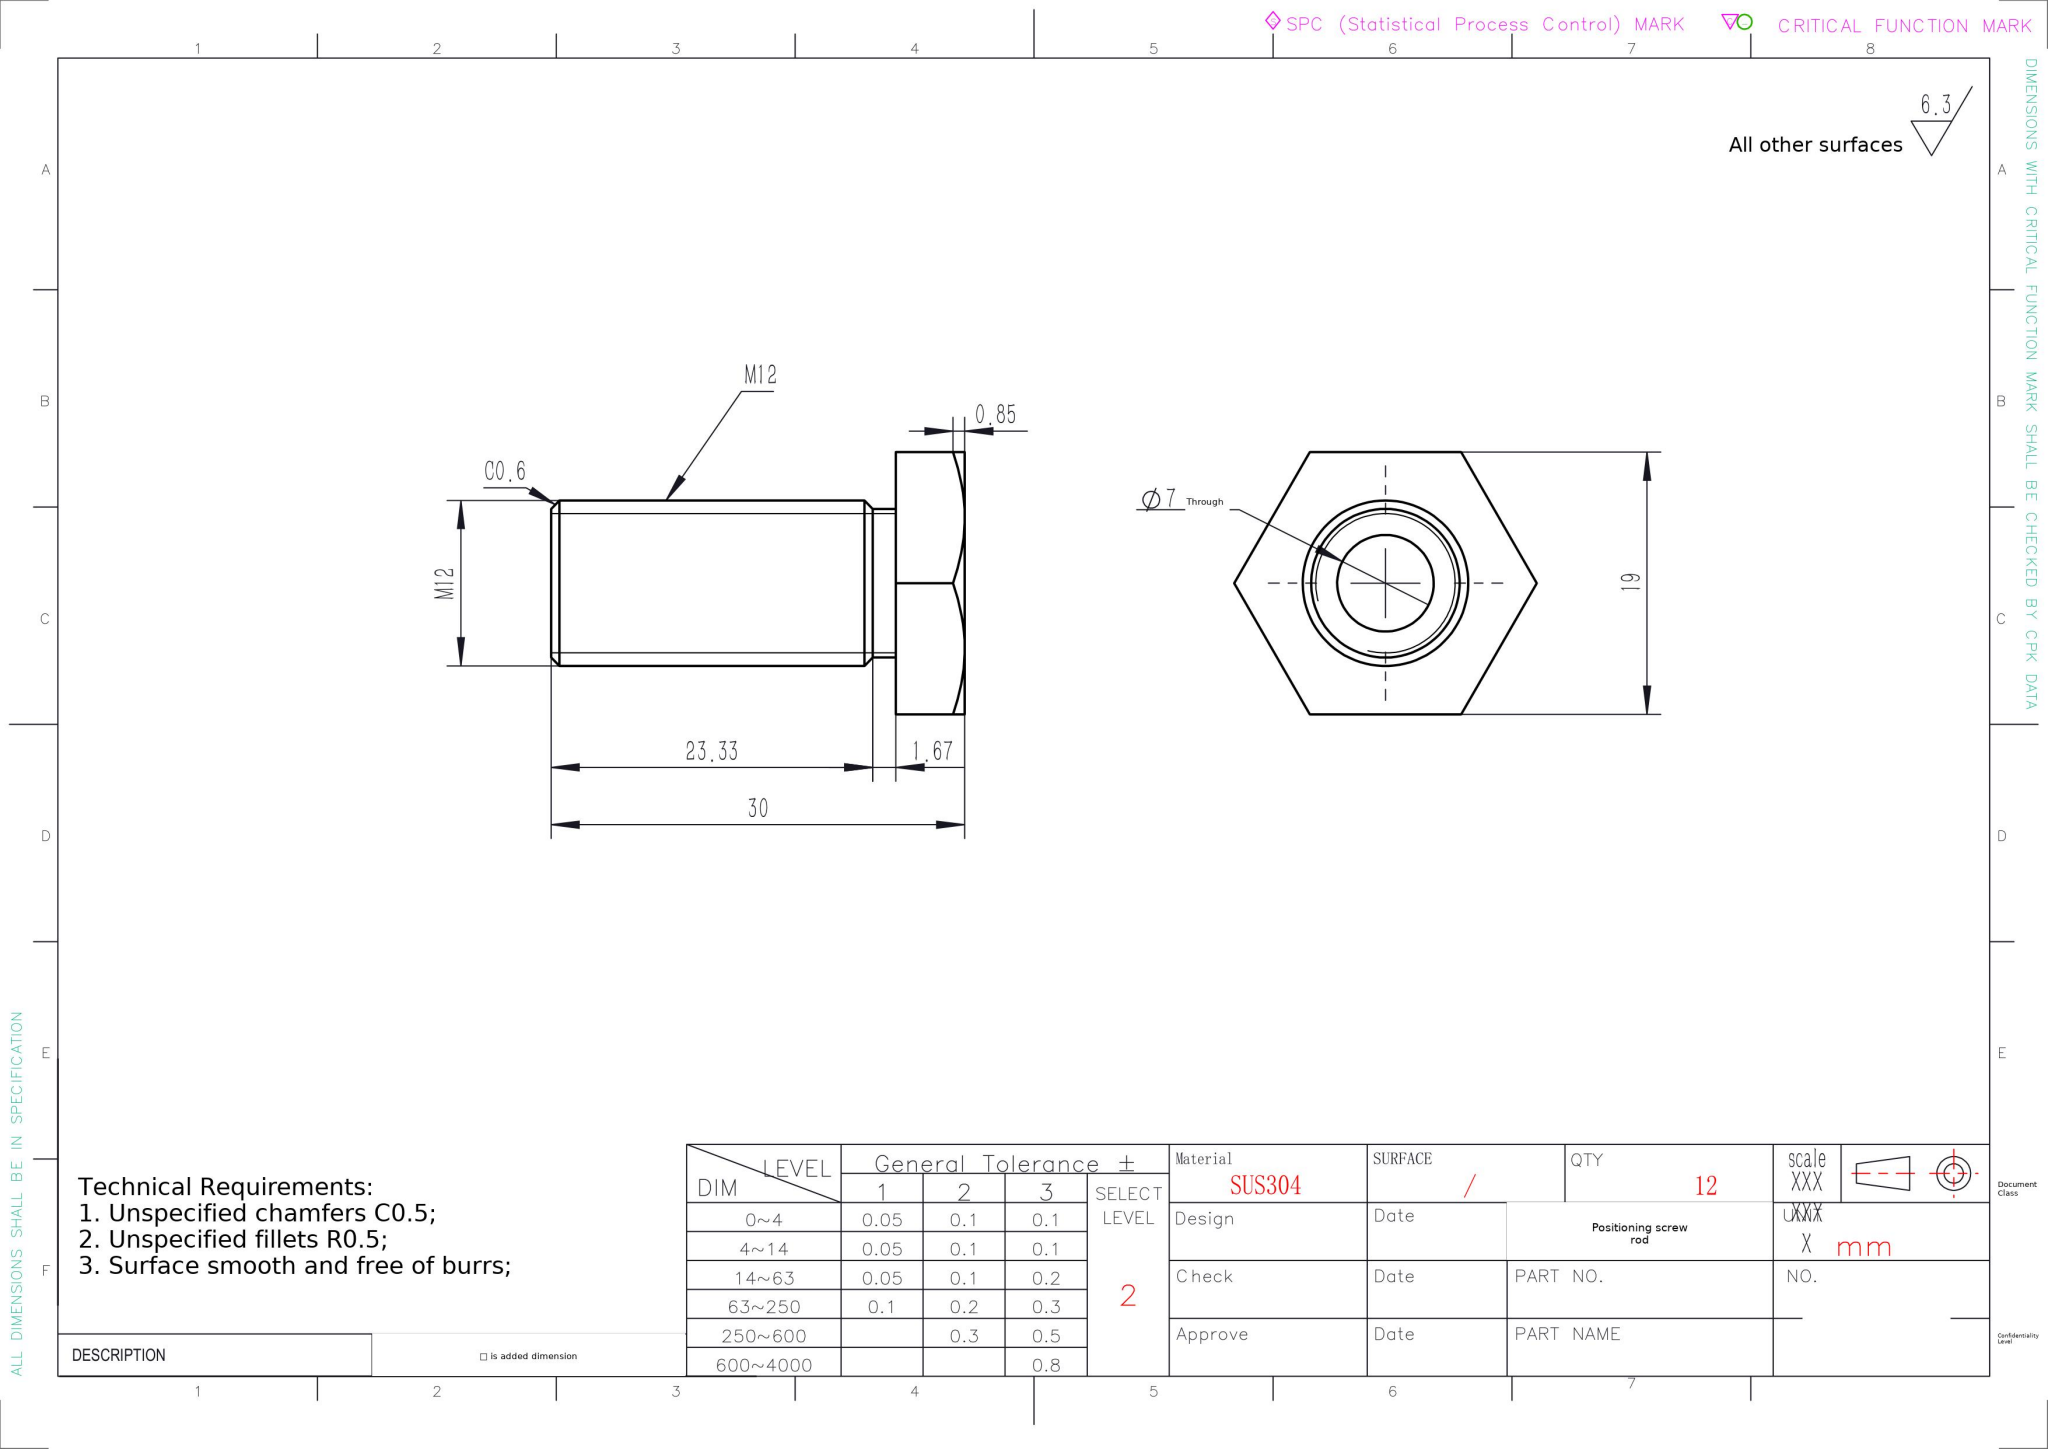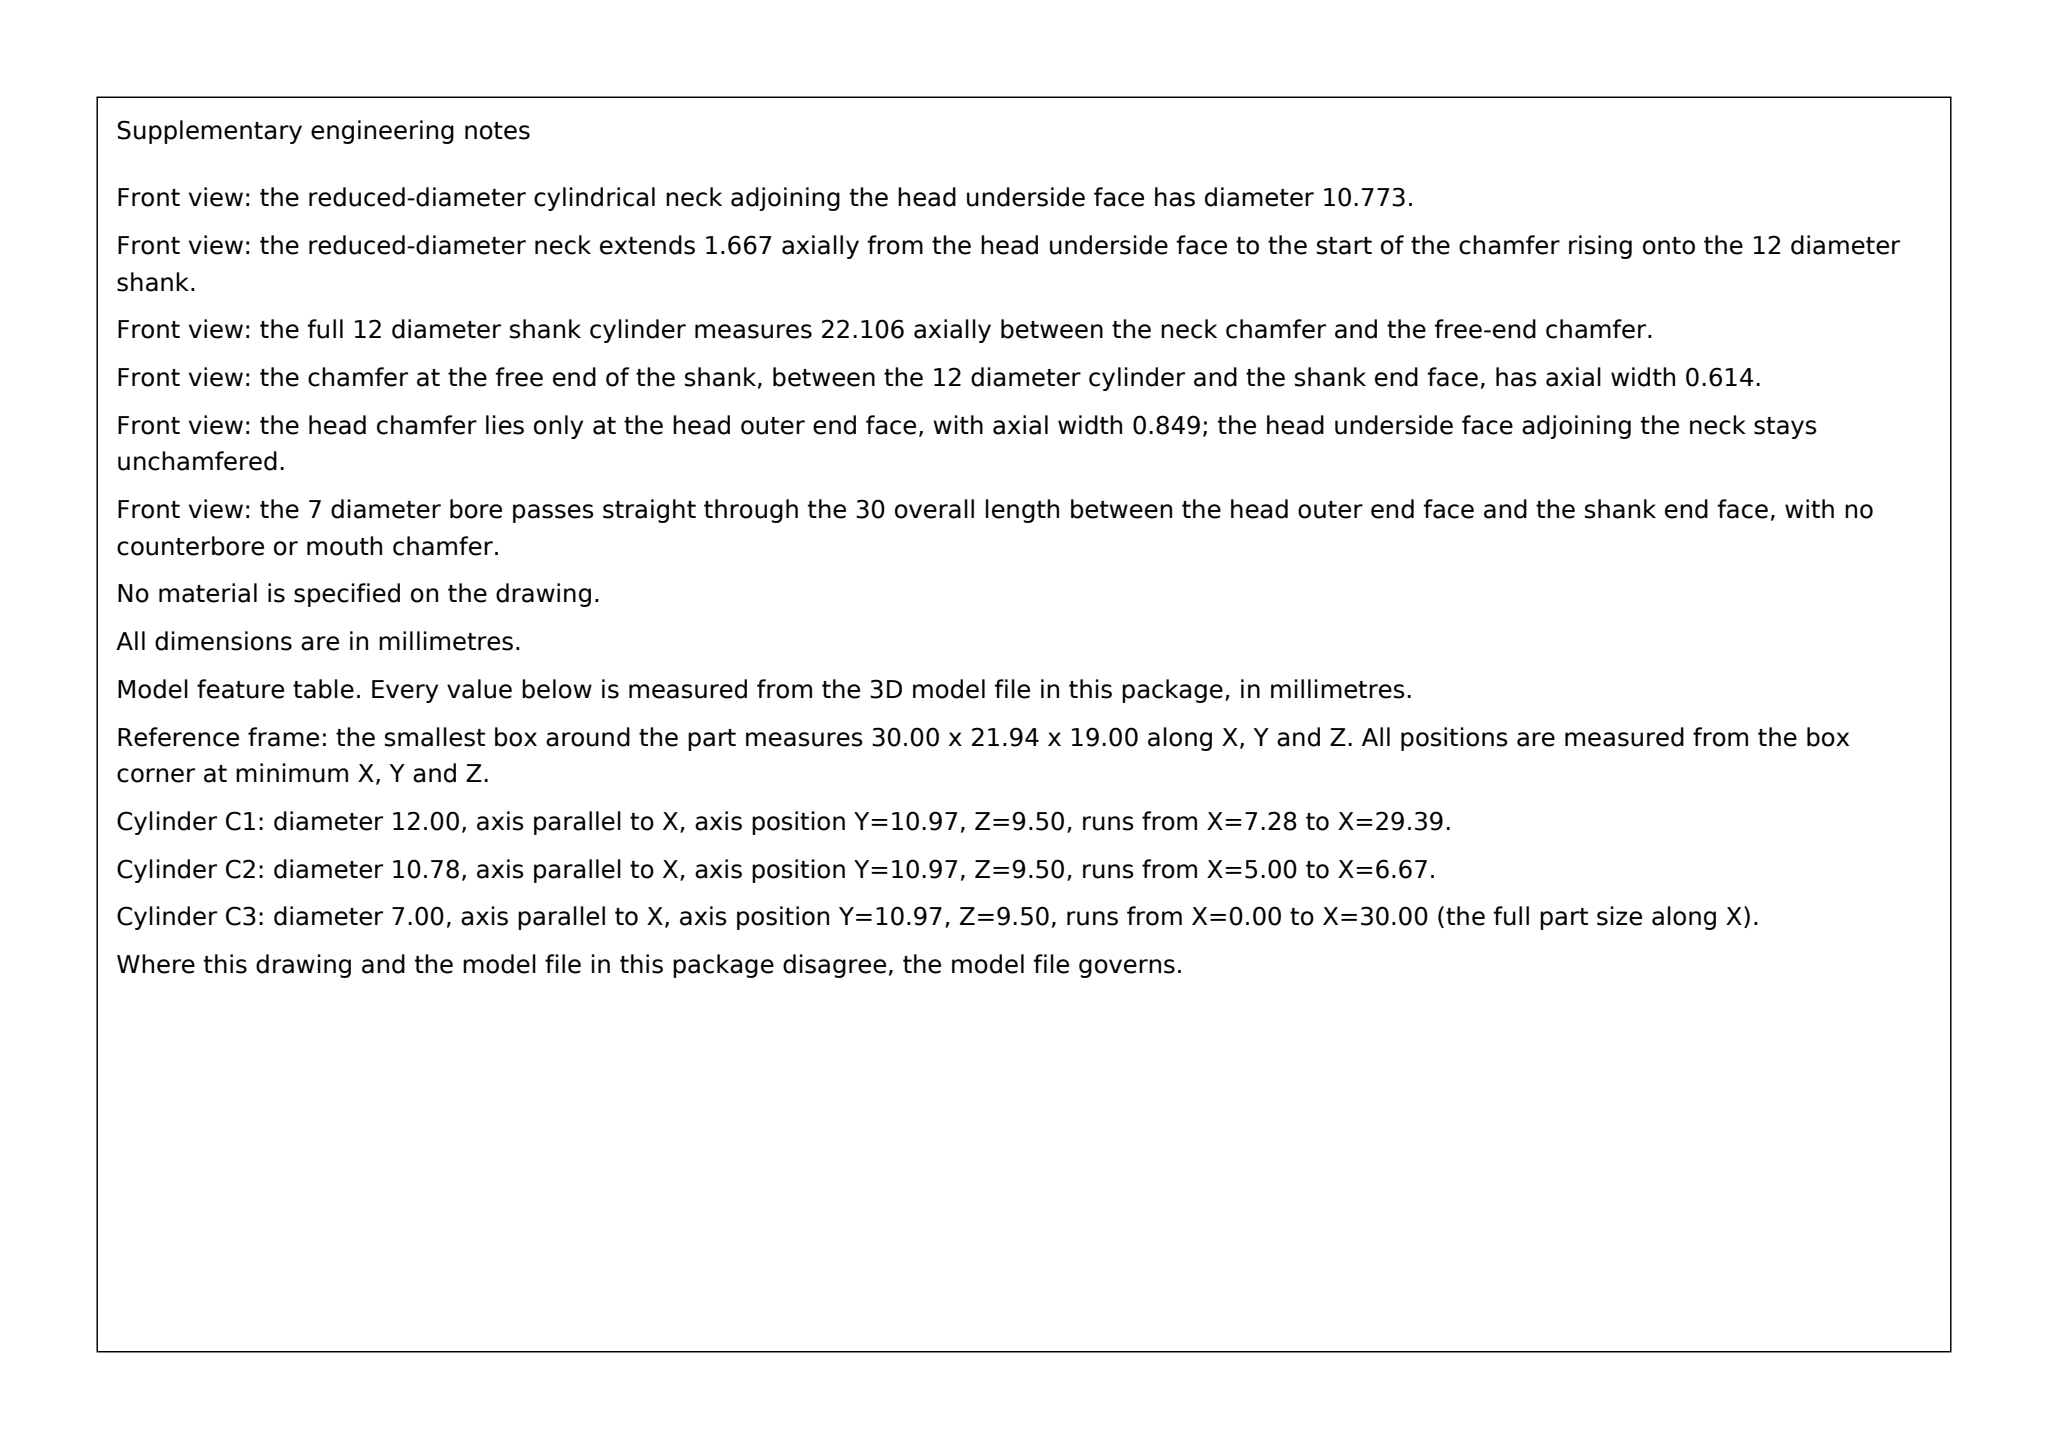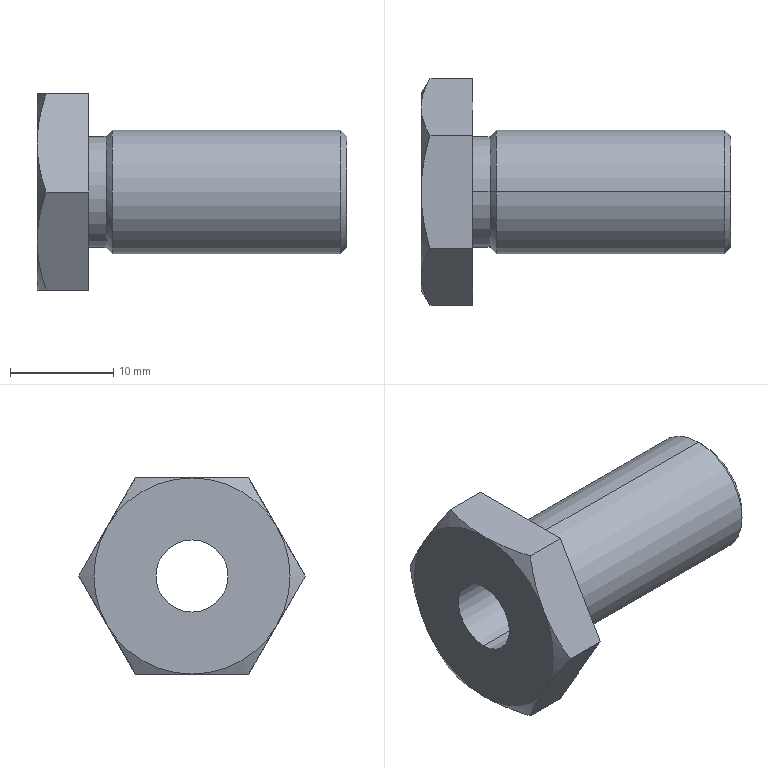Part | SolidWorks | mm | 1 solid | 25 faces | box 30 x 21.94 x 19 mm | volume 3178 mm3 | cone 10 | plane 9 | cylinder 6 | commonest cylinder face diameters 7 x2 12 x2 10.773 x2
Drawing notes:
HEX HD TOP CHAMFER 120° INCL x Ø15 (0.85 AXIAL) | from the solid: cones[included_angle,ref_dia]: [120.0, 15.0] x6 at hex head; 0.85 axial width shown
STEP:
#1=CARTESIAN_POINT('',(-5.,0.,3.5));
#2=VERTEX_POINT('',#1);
#3=CARTESIAN_POINT('',(-5.,0.,-3.5));
#4=VERTEX_POINT('',#3);
#5=CARTESIAN_POINT('',(-5.,0.,0.));
#6=DIRECTION('',(1.,0.,0.));
#7=DIRECTION('',(0.,0.,-1.));
#8=AXIS2_PLACEMENT_3D('',#5,#6,#7);
#9=CIRCLE('',#8,3.5);
#10=EDGE_CURVE('',#2,#4,#9,.T.);
#11=ORIENTED_EDGE('',*,*,#10,.F.);
#12=CARTESIAN_POINT('',(25.,0.,3.5));
#13=VERTEX_POINT('',#12);
#14=CARTESIAN_POINT('',(25.,0.,3.5));
#15=DIRECTION('',(1.,0.,0.));
#16=VECTOR('',#15,1000.);
#17=LINE('',#14,#16);
#18=EDGE_CURVE('',#2,#13,#17,.T.);
#19=ORIENTED_EDGE('',*,*,#18,.T.);
#20=CARTESIAN_POINT('',(25.,0.,-3.5));
#21=VERTEX_POINT('',#20);
#22=CARTESIAN_POINT('',(25.,0.,0.));
#23=DIRECTION('',(1.,0.,0.));
#24=DIRECTION('',(0.,0.,-1.));
#25=AXIS2_PLACEMENT_3D('',#22,#23,#24);
#26=CIRCLE('',#25,3.5);
#27=EDGE_CURVE('',#13,#21,#26,.T.);
#28=ORIENTED_EDGE('',*,*,#27,.T.);
#29=CARTESIAN_POINT('',(25.,0.,-3.5));
#30=DIRECTION('',(1.,0.,0.));
#31=VECTOR('',#30,1000.);
#32=LINE('',#29,#31);
#33=EDGE_CURVE('',#4,#21,#32,.T.);
#34=ORIENTED_EDGE('',*,*,#33,.F.);
#35=EDGE_LOOP('',(#11,#19,#28,#34));
#36=FACE_OUTER_BOUND('',#35,.T.);
#37=CARTESIAN_POINT('',(25.,0.,0.));
#38=DIRECTION('',(1.,0.,0.));
#39=DIRECTION('',(0.,0.,-1.));
#40=AXIS2_PLACEMENT_3D('',#37,#38,#39);
#41=CYLINDRICAL_SURFACE('',#40,3.5);
#42=ADVANCED_FACE('',(#36),#41,.F.);
#43=CARTESIAN_POINT('',(25.,0.,-5.386));
#44=VERTEX_POINT('',#43);
#45=CARTESIAN_POINT('',(25.,0.,5.386));
#46=VERTEX_POINT('',#45);
#47=CARTESIAN_POINT('',(25.,0.,0.));
#48=DIRECTION('',(1.,0.,0.));
#49=DIRECTION('',(0.,0.,-1.));
#50=AXIS2_PLACEMENT_3D('',#47,#48,#49);
#51=CIRCLE('',#50,5.386);
#52=EDGE_CURVE('',#44,#46,#51,.T.);
#53=ORIENTED_EDGE('',*,*,#52,.F.);
#54=CARTESIAN_POINT('',(24.386,0.,-6.));
#55=VERTEX_POINT('',#54);
#56=CARTESIAN_POINT('',(24.386,0.,-6.));
#57=DIRECTION('',(-0.7071,0.,-0.7071));
#58=VECTOR('',#57,1000.);
#59=LINE('',#56,#58);
#60=EDGE_CURVE('',#44,#55,#59,.T.);
#61=ORIENTED_EDGE('',*,*,#60,.T.);
#62=CARTESIAN_POINT('',(24.386,0.,6.));
#63=VERTEX_POINT('',#62);
#64=CARTESIAN_POINT('',(24.386,0.,0.));
#65=DIRECTION('',(1.,0.,0.));
#66=DIRECTION('',(0.,0.,-1.));
#67=AXIS2_PLACEMENT_3D('',#64,#65,#66);
#68=CIRCLE('',#67,6.);
#69=EDGE_CURVE('',#55,#63,#68,.T.);
#70=ORIENTED_EDGE('',*,*,#69,.T.);
#71=CARTESIAN_POINT('',(24.386,0.,6.));
#72=DIRECTION('',(-0.7071,0.,0.7071));
#73=VECTOR('',#72,1000.);
#74=LINE('',#71,#73);
#75=EDGE_CURVE('',#46,#63,#74,.T.);
#76=ORIENTED_EDGE('',*,*,#75,.F.);
#77=EDGE_LOOP('',(#53,#61,#70,#76));
#78=FACE_OUTER_BOUND('',#77,.T.);
#79=CARTESIAN_POINT('',(24.386,0.,0.));
#80=DIRECTION('',(-1.,0.,0.));
#81=DIRECTION('',(0.,0.,1.));
#82=AXIS2_PLACEMENT_3D('',#79,#80,#81);
#83=CONICAL_SURFACE('',#82,6.,0.7854);
#84=ADVANCED_FACE('',(#78),#83,.T.);
#85=CARTESIAN_POINT('',(2.28,0.,-6.));
#86=VERTEX_POINT('',#85);
#87=CARTESIAN_POINT('',(2.28,0.,6.));
#88=VERTEX_POINT('',#87);
#89=CARTESIAN_POINT('',(2.28,0.,0.));
#90=DIRECTION('',(1.,0.,0.));
#91=DIRECTION('',(0.,0.,-1.));
#92=AXIS2_PLACEMENT_3D('',#89,#90,#91);
#93=CIRCLE('',#92,6.);
#94=EDGE_CURVE('',#86,#88,#93,.T.);
#95=ORIENTED_EDGE('',*,*,#94,.T.);
#96=CARTESIAN_POINT('',(25.,0.,6.));
#97=DIRECTION('',(1.,0.,0.));
#98=VECTOR('',#97,1000.);
#99=LINE('',#96,#98);
#100=EDGE_CURVE('',#88,#63,#99,.T.);
#101=ORIENTED_EDGE('',*,*,#100,.T.);
#102=ORIENTED_EDGE('',*,*,#69,.F.);
#103=CARTESIAN_POINT('',(25.,0.,-6.));
#104=DIRECTION('',(1.,0.,0.));
#105=VECTOR('',#104,1000.);
#106=LINE('',#103,#105);
#107=EDGE_CURVE('',#86,#55,#106,.T.);
#108=ORIENTED_EDGE('',*,*,#107,.F.);
#109=EDGE_LOOP('',(#95,#101,#102,#108));
#110=FACE_OUTER_BOUND('',#109,.T.);
#111=CARTESIAN_POINT('',(25.,0.,0.));
#112=DIRECTION('',(1.,0.,0.));
#113=DIRECTION('',(0.,0.,-1.));
#114=AXIS2_PLACEMENT_3D('',#111,#112,#113);
#115=CYLINDRICAL_SURFACE('',#114,6.);
#116=ADVANCED_FACE('',(#110),#115,.T.);
#117=CARTESIAN_POINT('',(1.667,0.,-5.386));
#118=VERTEX_POINT('',#117);
#119=CARTESIAN_POINT('',(1.667,0.,5.386));
#120=VERTEX_POINT('',#119);
#121=CARTESIAN_POINT('',(1.667,0.,0.));
#122=DIRECTION('',(1.,0.,0.));
#123=DIRECTION('',(0.,0.,-1.));
#124=AXIS2_PLACEMENT_3D('',#121,#122,#123);
#125=CIRCLE('',#124,5.386);
#126=EDGE_CURVE('',#118,#120,#125,.T.);
#127=ORIENTED_EDGE('',*,*,#126,.T.);
#128=CARTESIAN_POINT('',(1.667,0.,5.386));
#129=DIRECTION('',(0.7071,0.,0.7071));
#130=VECTOR('',#129,1000.);
#131=LINE('',#128,#130);
#132=EDGE_CURVE('',#120,#88,#131,.T.);
#133=ORIENTED_EDGE('',*,*,#132,.T.);
#134=ORIENTED_EDGE('',*,*,#94,.F.);
#135=CARTESIAN_POINT('',(1.667,0.,-5.386));
#136=DIRECTION('',(0.7071,0.,-0.7071));
#137=VECTOR('',#136,1000.);
#138=LINE('',#135,#137);
#139=EDGE_CURVE('',#118,#86,#138,.T.);
#140=ORIENTED_EDGE('',*,*,#139,.F.);
#141=EDGE_LOOP('',(#127,#133,#134,#140));
#142=FACE_OUTER_BOUND('',#141,.T.);
#143=CARTESIAN_POINT('',(1.667,0.,0.));
#144=DIRECTION('',(1.,0.,0.));
#145=DIRECTION('',(0.,0.,-1.));
#146=AXIS2_PLACEMENT_3D('',#143,#144,#145);
#147=CONICAL_SURFACE('',#146,5.386,0.7854);
#148=ADVANCED_FACE('',(#142),#147,.T.);
#149=CARTESIAN_POINT('',(0.,0.,-5.386));
#150=VERTEX_POINT('',#149);
#151=CARTESIAN_POINT('',(0.,0.,5.386));
#152=VERTEX_POINT('',#151);
#153=CARTESIAN_POINT('',(0.,0.,0.));
#154=DIRECTION('',(1.,0.,0.));
#155=DIRECTION('',(0.,0.,-1.));
#156=AXIS2_PLACEMENT_3D('',#153,#154,#155);
#157=CIRCLE('',#156,5.386);
#158=EDGE_CURVE('',#150,#152,#157,.T.);
#159=ORIENTED_EDGE('',*,*,#158,.T.);
#160=CARTESIAN_POINT('',(25.,0.,5.386));
#161=DIRECTION('',(1.,0.,0.));
#162=VECTOR('',#161,1000.);
#163=LINE('',#160,#162);
#164=EDGE_CURVE('',#152,#120,#163,.T.);
#165=ORIENTED_EDGE('',*,*,#164,.T.);
#166=ORIENTED_EDGE('',*,*,#126,.F.);
#167=CARTESIAN_POINT('',(25.,0.,-5.386));
#168=DIRECTION('',(1.,0.,0.));
#169=VECTOR('',#168,1000.);
#170=LINE('',#167,#169);
#171=EDGE_CURVE('',#150,#118,#170,.T.);
#172=ORIENTED_EDGE('',*,*,#171,.F.);
#173=EDGE_LOOP('',(#159,#165,#166,#172));
#174=FACE_OUTER_BOUND('',#173,.T.);
#175=CARTESIAN_POINT('',(25.,0.,0.));
#176=DIRECTION('',(1.,0.,0.));
#177=DIRECTION('',(0.,0.,-1.));
#178=AXIS2_PLACEMENT_3D('',#175,#176,#177);
#179=CYLINDRICAL_SURFACE('',#178,5.386);
#180=ADVANCED_FACE('',(#174),#179,.T.);
#181=ORIENTED_EDGE('',*,*,#164,.F.);
#182=CARTESIAN_POINT('',(0.,0.,0.));
#183=DIRECTION('',(1.,0.,0.));
#184=DIRECTION('',(0.,0.,-1.));
#185=AXIS2_PLACEMENT_3D('',#182,#183,#184);
#186=CIRCLE('',#185,5.386);
#187=EDGE_CURVE('',#152,#150,#186,.T.);
#188=ORIENTED_EDGE('',*,*,#187,.T.);
#189=ORIENTED_EDGE('',*,*,#171,.T.);
#190=CARTESIAN_POINT('',(1.667,0.,0.));
#191=DIRECTION('',(1.,0.,0.));
#192=DIRECTION('',(0.,0.,-1.));
#193=AXIS2_PLACEMENT_3D('',#190,#191,#192);
#194=CIRCLE('',#193,5.386);
#195=EDGE_CURVE('',#120,#118,#194,.T.);
#196=ORIENTED_EDGE('',*,*,#195,.F.);
#197=EDGE_LOOP('',(#181,#188,#189,#196));
#198=FACE_OUTER_BOUND('',#197,.T.);
#199=CARTESIAN_POINT('',(25.,0.,0.));
#200=DIRECTION('',(1.,0.,0.));
#201=DIRECTION('',(0.,0.,-1.));
#202=AXIS2_PLACEMENT_3D('',#199,#200,#201);
#203=CYLINDRICAL_SURFACE('',#202,5.386);
#204=ADVANCED_FACE('',(#198),#203,.T.);
#205=ORIENTED_EDGE('',*,*,#132,.F.);
#206=ORIENTED_EDGE('',*,*,#195,.T.);
#207=ORIENTED_EDGE('',*,*,#139,.T.);
#208=CARTESIAN_POINT('',(2.28,0.,0.));
#209=DIRECTION('',(1.,0.,0.));
#210=DIRECTION('',(0.,0.,-1.));
#211=AXIS2_PLACEMENT_3D('',#208,#209,#210);
#212=CIRCLE('',#211,6.);
#213=EDGE_CURVE('',#88,#86,#212,.T.);
#214=ORIENTED_EDGE('',*,*,#213,.F.);
#215=EDGE_LOOP('',(#205,#206,#207,#214));
#216=FACE_OUTER_BOUND('',#215,.T.);
#217=CARTESIAN_POINT('',(1.667,0.,0.));
#218=DIRECTION('',(1.,0.,0.));
#219=DIRECTION('',(0.,0.,-1.));
#220=AXIS2_PLACEMENT_3D('',#217,#218,#219);
#221=CONICAL_SURFACE('',#220,5.386,0.7854);
#222=ADVANCED_FACE('',(#216),#221,.T.);
#223=ORIENTED_EDGE('',*,*,#100,.F.);
#224=ORIENTED_EDGE('',*,*,#213,.T.);
#225=ORIENTED_EDGE('',*,*,#107,.T.);
#226=CARTESIAN_POINT('',(24.386,0.,0.));
#227=DIRECTION('',(1.,0.,0.));
#228=DIRECTION('',(0.,0.,-1.));
#229=AXIS2_PLACEMENT_3D('',#226,#227,#228);
#230=CIRCLE('',#229,6.);
#231=EDGE_CURVE('',#63,#55,#230,.T.);
#232=ORIENTED_EDGE('',*,*,#231,.F.);
#233=EDGE_LOOP('',(#223,#224,#225,#232));
#234=FACE_OUTER_BOUND('',#233,.T.);
#235=CARTESIAN_POINT('',(25.,0.,0.));
#236=DIRECTION('',(1.,0.,0.));
#237=DIRECTION('',(0.,0.,-1.));
#238=AXIS2_PLACEMENT_3D('',#235,#236,#237);
#239=CYLINDRICAL_SURFACE('',#238,6.);
#240=ADVANCED_FACE('',(#234),#239,.T.);
#241=ORIENTED_EDGE('',*,*,#60,.F.);
#242=CARTESIAN_POINT('',(25.,0.,0.));
#243=DIRECTION('',(1.,0.,0.));
#244=DIRECTION('',(0.,0.,-1.));
#245=AXIS2_PLACEMENT_3D('',#242,#243,#244);
#246=CIRCLE('',#245,5.386);
#247=EDGE_CURVE('',#46,#44,#246,.T.);
#248=ORIENTED_EDGE('',*,*,#247,.F.);
#249=ORIENTED_EDGE('',*,*,#75,.T.);
#250=ORIENTED_EDGE('',*,*,#231,.T.);
#251=EDGE_LOOP('',(#241,#248,#249,#250));
#252=FACE_OUTER_BOUND('',#251,.T.);
#253=CARTESIAN_POINT('',(24.386,0.,0.));
#254=DIRECTION('',(-1.,0.,0.));
#255=DIRECTION('',(0.,0.,1.));
#256=AXIS2_PLACEMENT_3D('',#253,#254,#255);
#257=CONICAL_SURFACE('',#256,6.,0.7854);
#258=ADVANCED_FACE('',(#252),#257,.T.);
#259=CARTESIAN_POINT('',(25.,0.,0.));
#260=DIRECTION('',(1.,0.,0.));
#261=DIRECTION('',(0.,0.,-1.));
#262=AXIS2_PLACEMENT_3D('',#259,#260,#261);
#263=CIRCLE('',#262,3.5);
#264=EDGE_CURVE('',#21,#13,#263,.T.);
#265=ORIENTED_EDGE('',*,*,#264,.F.);
#266=ORIENTED_EDGE('',*,*,#27,.F.);
#267=EDGE_LOOP('',(#265,#266));
#268=FACE_BOUND('',#267,.T.);
#269=ORIENTED_EDGE('',*,*,#247,.T.);
#270=ORIENTED_EDGE('',*,*,#52,.T.);
#271=EDGE_LOOP('',(#269,#270));
#272=FACE_OUTER_BOUND('',#271,.T.);
#273=CARTESIAN_POINT('',(25.,5.386,0.));
#274=DIRECTION('',(-1.,0.,0.));
#275=DIRECTION('',(0.,0.,1.));
#276=AXIS2_PLACEMENT_3D('',#273,#274,#275);
#277=PLANE('',#276);
#278=ADVANCED_FACE('',(#268,#272),#277,.F.);
#279=CARTESIAN_POINT('',(-4.151,-5.485,9.5));
#280=VERTEX_POINT('',#279);
#281=CARTESIAN_POINT('',(-5.,0.,9.5));
#282=VERTEX_POINT('',#281);
#283=CARTESIAN_POINT('',(-4.151,-5.485,9.5));
#284=CARTESIAN_POINT('',(-4.409,-4.592,9.5));
#285=CARTESIAN_POINT('',(-4.625,-3.679,9.5));
#286=CARTESIAN_POINT('',(-4.92,-1.848,9.5));
#287=CARTESIAN_POINT('',(-5.,-0.9276,9.5));
#288=CARTESIAN_POINT('',(-5.,0.,9.5));
#289=B_SPLINE_CURVE_WITH_KNOTS('',3,(#283,#284,#285,#286,#287,#288),.UNSPECIFIED.,.F.,.F.,(4,2,4),(0.01004,0.01282,0.01559),.UNSPECIFIED.);
#290=EDGE_CURVE('',#280,#282,#289,.T.);
#291=ORIENTED_EDGE('',*,*,#290,.F.);
#292=CARTESIAN_POINT('',(0.,-5.485,9.5));
#293=VERTEX_POINT('',#292);
#294=CARTESIAN_POINT('',(-5.,-5.485,9.5));
#295=DIRECTION('',(1.,0.,0.));
#296=VECTOR('',#295,1000.);
#297=LINE('',#294,#296);
#298=EDGE_CURVE('',#280,#293,#297,.T.);
#299=ORIENTED_EDGE('',*,*,#298,.T.);
#300=CARTESIAN_POINT('',(0.,5.485,9.5));
#301=VERTEX_POINT('',#300);
#302=CARTESIAN_POINT('',(0.,5.485,9.5));
#303=DIRECTION('',(0.,-1.,0.));
#304=VECTOR('',#303,1000.);
#305=LINE('',#302,#304);
#306=EDGE_CURVE('',#301,#293,#305,.T.);
#307=ORIENTED_EDGE('',*,*,#306,.F.);
#308=CARTESIAN_POINT('',(-4.151,5.485,9.5));
#309=VERTEX_POINT('',#308);
#310=CARTESIAN_POINT('',(-5.,5.485,9.5));
#311=DIRECTION('',(1.,0.,0.));
#312=VECTOR('',#311,1000.);
#313=LINE('',#310,#312);
#314=EDGE_CURVE('',#309,#301,#313,.T.);
#315=ORIENTED_EDGE('',*,*,#314,.F.);
#316=CARTESIAN_POINT('',(-5.,0.,9.5));
#317=CARTESIAN_POINT('',(-5.,0.4641,9.5));
#318=CARTESIAN_POINT('',(-4.98,0.9304,9.5));
#319=CARTESIAN_POINT('',(-4.902,1.864,9.5));
#320=CARTESIAN_POINT('',(-4.844,2.326,9.5));
#321=CARTESIAN_POINT('',(-4.621,3.699,9.5));
#322=CARTESIAN_POINT('',(-4.408,4.598,9.5));
#323=CARTESIAN_POINT('',(-4.151,5.485,9.5));
#324=B_SPLINE_CURVE_WITH_KNOTS('',3,(#316,#317,#318,#319,#320,#321,#322,#323),.UNSPECIFIED.,.F.,.F.,(4,2,2,4),(0.01559,0.01698,0.01837,0.02115),.UNSPECIFIED.);
#325=EDGE_CURVE('',#282,#309,#324,.T.);
#326=ORIENTED_EDGE('',*,*,#325,.F.);
#327=EDGE_LOOP('',(#291,#299,#307,#315,#326));
#328=FACE_OUTER_BOUND('',#327,.T.);
#329=CARTESIAN_POINT('',(-5.,5.485,9.5));
#330=DIRECTION('',(0.,0.,1.));
#331=DIRECTION('',(1.,0.,0.));
#332=AXIS2_PLACEMENT_3D('',#329,#330,#331);
#333=PLANE('',#332);
#334=ADVANCED_FACE('',(#328),#333,.T.);
#335=CARTESIAN_POINT('',(-4.151,-10.97,-0.));
#336=VERTEX_POINT('',#335);
#337=CARTESIAN_POINT('',(-5.,-8.227,4.75));
#338=VERTEX_POINT('',#337);
#339=CARTESIAN_POINT('',(-4.151,-10.97,-0.));
#340=CARTESIAN_POINT('',(-4.411,-10.521,0.777));
#341=CARTESIAN_POINT('',(-4.624,-10.069,1.56));
#342=CARTESIAN_POINT('',(-4.919,-9.156,3.142));
#343=CARTESIAN_POINT('',(-5.,-8.694,3.941));
#344=CARTESIAN_POINT('',(-5.,-8.227,4.75));
#345=B_SPLINE_CURVE_WITH_KNOTS('',3,(#339,#340,#341,#342,#343,#344),.UNSPECIFIED.,.F.,.F.,(4,2,4),(0.00000024,0.002775,0.00555),.UNSPECIFIED.);
#346=EDGE_CURVE('',#336,#338,#345,.T.);
#347=ORIENTED_EDGE('',*,*,#346,.F.);
#348=CARTESIAN_POINT('',(0.,-10.97,0.));
#349=VERTEX_POINT('',#348);
#350=CARTESIAN_POINT('',(-5.,-10.97,0.));
#351=DIRECTION('',(1.,0.,0.));
#352=VECTOR('',#351,1000.);
#353=LINE('',#350,#352);
#354=EDGE_CURVE('',#336,#349,#353,.T.);
#355=ORIENTED_EDGE('',*,*,#354,.T.);
#356=CARTESIAN_POINT('',(0.,-5.485,9.5));
#357=DIRECTION('',(0.,-0.5,-0.866));
#358=VECTOR('',#357,1000.);
#359=LINE('',#356,#358);
#360=EDGE_CURVE('',#293,#349,#359,.T.);
#361=ORIENTED_EDGE('',*,*,#360,.F.);
#362=ORIENTED_EDGE('',*,*,#298,.F.);
#363=CARTESIAN_POINT('',(-5.,-8.227,4.75));
#364=CARTESIAN_POINT('',(-5.,-7.995,5.153));
#365=CARTESIAN_POINT('',(-4.98,-7.761,5.558));
#366=CARTESIAN_POINT('',(-4.902,-7.298,6.359));
#367=CARTESIAN_POINT('',(-4.845,-7.069,6.757));
#368=CARTESIAN_POINT('',(-4.623,-6.384,7.943));
#369=CARTESIAN_POINT('',(-4.41,-5.932,8.725));
#370=CARTESIAN_POINT('',(-4.151,-5.485,9.5));
#371=B_SPLINE_CURVE_WITH_KNOTS('',3,(#363,#364,#365,#366,#367,#368,#369,#370),.UNSPECIFIED.,.F.,.F.,(4,2,2,4),(0.00555,0.006932,0.008314,0.01108),.UNSPECIFIED.);
#372=EDGE_CURVE('',#338,#280,#371,.T.);
#373=ORIENTED_EDGE('',*,*,#372,.F.);
#374=EDGE_LOOP('',(#347,#355,#361,#362,#373));
#375=FACE_OUTER_BOUND('',#374,.T.);
#376=CARTESIAN_POINT('',(-5.,-5.485,9.5));
#377=DIRECTION('',(0.,-0.866,0.5));
#378=DIRECTION('',(0.,-0.5,-0.866));
#379=AXIS2_PLACEMENT_3D('',#376,#377,#378);
#380=PLANE('',#379);
#381=ADVANCED_FACE('',(#375),#380,.T.);
#382=CARTESIAN_POINT('',(-4.151,-5.485,-9.5));
#383=VERTEX_POINT('',#382);
#384=CARTESIAN_POINT('',(-5.,-8.227,-4.75));
#385=VERTEX_POINT('',#384);
#386=CARTESIAN_POINT('',(-4.151,-5.485,-9.5));
#387=CARTESIAN_POINT('',(-4.411,-5.933,-8.723));
#388=CARTESIAN_POINT('',(-4.624,-6.385,-7.94));
#389=CARTESIAN_POINT('',(-4.919,-7.299,-6.358));
#390=CARTESIAN_POINT('',(-5.,-7.76,-5.559));
#391=CARTESIAN_POINT('',(-5.,-8.227,-4.75));
#392=B_SPLINE_CURVE_WITH_KNOTS('',3,(#386,#387,#388,#389,#390,#391),.UNSPECIFIED.,.F.,.F.,(4,2,4),(0.00000024,0.002775,0.00555),.UNSPECIFIED.);
#393=EDGE_CURVE('',#383,#385,#392,.T.);
#394=ORIENTED_EDGE('',*,*,#393,.F.);
#395=CARTESIAN_POINT('',(0.,-5.485,-9.5));
#396=VERTEX_POINT('',#395);
#397=CARTESIAN_POINT('',(-5.,-5.485,-9.5));
#398=DIRECTION('',(1.,0.,0.));
#399=VECTOR('',#398,1000.);
#400=LINE('',#397,#399);
#401=EDGE_CURVE('',#383,#396,#400,.T.);
#402=ORIENTED_EDGE('',*,*,#401,.T.);
#403=CARTESIAN_POINT('',(0.,-10.97,0.));
#404=DIRECTION('',(0.,0.5,-0.866));
#405=VECTOR('',#404,1000.);
#406=LINE('',#403,#405);
#407=EDGE_CURVE('',#349,#396,#406,.T.);
#408=ORIENTED_EDGE('',*,*,#407,.F.);
#409=ORIENTED_EDGE('',*,*,#354,.F.);
#410=CARTESIAN_POINT('',(-5.,-8.227,-4.75));
#411=CARTESIAN_POINT('',(-5.,-8.46,-4.347));
#412=CARTESIAN_POINT('',(-4.98,-8.694,-3.942));
#413=CARTESIAN_POINT('',(-4.902,-9.156,-3.141));
#414=CARTESIAN_POINT('',(-4.845,-9.386,-2.743));
#415=CARTESIAN_POINT('',(-4.623,-10.071,-1.557));
#416=CARTESIAN_POINT('',(-4.41,-10.522,-0.7751));
#417=CARTESIAN_POINT('',(-4.151,-10.97,-0.));
#418=B_SPLINE_CURVE_WITH_KNOTS('',3,(#410,#411,#412,#413,#414,#415,#416,#417),.UNSPECIFIED.,.F.,.F.,(4,2,2,4),(0.00555,0.006932,0.008314,0.01108),.UNSPECIFIED.);
#419=EDGE_CURVE('',#385,#336,#418,.T.);
#420=ORIENTED_EDGE('',*,*,#419,.F.);
#421=EDGE_LOOP('',(#394,#402,#408,#409,#420));
#422=FACE_OUTER_BOUND('',#421,.T.);
#423=CARTESIAN_POINT('',(-5.,-10.97,0.));
#424=DIRECTION('',(0.,-0.866,-0.5));
#425=DIRECTION('',(0.,0.5,-0.866));
#426=AXIS2_PLACEMENT_3D('',#423,#424,#425);
#427=PLANE('',#426);
#428=ADVANCED_FACE('',(#422),#427,.T.);
#429=CARTESIAN_POINT('',(-4.151,5.485,-9.5));
#430=VERTEX_POINT('',#429);
#431=CARTESIAN_POINT('',(-5.,0.,-9.5));
#432=VERTEX_POINT('',#431);
#433=CARTESIAN_POINT('',(-4.151,5.485,-9.5));
#434=CARTESIAN_POINT('',(-4.408,4.598,-9.5));
#435=CARTESIAN_POINT('',(-4.621,3.699,-9.5));
#436=CARTESIAN_POINT('',(-4.844,2.326,-9.5));
#437=CARTESIAN_POINT('',(-4.902,1.864,-9.5));
#438=CARTESIAN_POINT('',(-4.98,0.9304,-9.5));
#439=CARTESIAN_POINT('',(-5.,0.4641,-9.5));
#440=CARTESIAN_POINT('',(-5.,0.,-9.5));
#441=B_SPLINE_CURVE_WITH_KNOTS('',3,(#433,#434,#435,#436,#437,#438,#439,#440),.UNSPECIFIED.,.F.,.F.,(4,2,2,4),(0.02794,0.03072,0.03211,0.0335),.UNSPECIFIED.);
#442=EDGE_CURVE('',#430,#432,#441,.T.);
#443=ORIENTED_EDGE('',*,*,#442,.F.);
#444=CARTESIAN_POINT('',(0.,5.485,-9.5));
#445=VERTEX_POINT('',#444);
#446=CARTESIAN_POINT('',(-5.,5.485,-9.5));
#447=DIRECTION('',(1.,0.,0.));
#448=VECTOR('',#447,1000.);
#449=LINE('',#446,#448);
#450=EDGE_CURVE('',#430,#445,#449,.T.);
#451=ORIENTED_EDGE('',*,*,#450,.T.);
#452=CARTESIAN_POINT('',(0.,-5.485,-9.5));
#453=DIRECTION('',(0.,1.,0.));
#454=VECTOR('',#453,1000.);
#455=LINE('',#452,#454);
#456=EDGE_CURVE('',#396,#445,#455,.T.);
#457=ORIENTED_EDGE('',*,*,#456,.F.);
#458=ORIENTED_EDGE('',*,*,#401,.F.);
#459=CARTESIAN_POINT('',(-5.,0.,-9.5));
#460=CARTESIAN_POINT('',(-5.,-0.9276,-9.5));
#461=CARTESIAN_POINT('',(-4.92,-1.848,-9.5));
#462=CARTESIAN_POINT('',(-4.625,-3.679,-9.5));
#463=CARTESIAN_POINT('',(-4.409,-4.592,-9.5));
#464=CARTESIAN_POINT('',(-4.151,-5.485,-9.5));
#465=B_SPLINE_CURVE_WITH_KNOTS('',3,(#459,#460,#461,#462,#463,#464),.UNSPECIFIED.,.F.,.F.,(4,2,4),(0.0335,0.03627,0.03905),.UNSPECIFIED.);
#466=EDGE_CURVE('',#432,#383,#465,.T.);
#467=ORIENTED_EDGE('',*,*,#466,.F.);
#468=EDGE_LOOP('',(#443,#451,#457,#458,#467));
#469=FACE_OUTER_BOUND('',#468,.T.);
#470=CARTESIAN_POINT('',(-5.,-5.485,-9.5));
#471=DIRECTION('',(0.,0.,-1.));
#472=DIRECTION('',(-1.,0.,0.));
#473=AXIS2_PLACEMENT_3D('',#470,#471,#472);
#474=PLANE('',#473);
#475=ADVANCED_FACE('',(#469),#474,.T.);
#476=CARTESIAN_POINT('',(-4.151,10.97,0.));
#477=VERTEX_POINT('',#476);
#478=CARTESIAN_POINT('',(-5.,8.227,-4.75));
#479=VERTEX_POINT('',#478);
#480=CARTESIAN_POINT('',(-4.151,10.97,0.));
#481=CARTESIAN_POINT('',(-4.411,10.521,-0.777));
#482=CARTESIAN_POINT('',(-4.624,10.069,-1.56));
#483=CARTESIAN_POINT('',(-4.919,9.156,-3.142));
#484=CARTESIAN_POINT('',(-5.,8.694,-3.941));
#485=CARTESIAN_POINT('',(-5.,8.227,-4.75));
#486=B_SPLINE_CURVE_WITH_KNOTS('',3,(#480,#481,#482,#483,#484,#485),.UNSPECIFIED.,.F.,.F.,(4,2,4),(0.00000024,0.002775,0.00555),.UNSPECIFIED.);
#487=EDGE_CURVE('',#477,#479,#486,.T.);
#488=ORIENTED_EDGE('',*,*,#487,.F.);
#489=CARTESIAN_POINT('',(0.,10.97,0.));
#490=VERTEX_POINT('',#489);
#491=CARTESIAN_POINT('',(-5.,10.97,0.));
#492=DIRECTION('',(1.,0.,0.));
#493=VECTOR('',#492,1000.);
#494=LINE('',#491,#493);
#495=EDGE_CURVE('',#477,#490,#494,.T.);
#496=ORIENTED_EDGE('',*,*,#495,.T.);
#497=CARTESIAN_POINT('',(0.,5.485,-9.5));
#498=DIRECTION('',(0.,0.5,0.866));
#499=VECTOR('',#498,1000.);
#500=LINE('',#497,#499);
#501=EDGE_CURVE('',#445,#490,#500,.T.);
#502=ORIENTED_EDGE('',*,*,#501,.F.);
#503=ORIENTED_EDGE('',*,*,#450,.F.);
#504=CARTESIAN_POINT('',(-5.,8.227,-4.75));
#505=CARTESIAN_POINT('',(-5.,7.995,-5.153));
#506=CARTESIAN_POINT('',(-4.98,7.761,-5.558));
#507=CARTESIAN_POINT('',(-4.902,7.298,-6.359));
#508=CARTESIAN_POINT('',(-4.845,7.069,-6.757));
#509=CARTESIAN_POINT('',(-4.623,6.384,-7.943));
#510=CARTESIAN_POINT('',(-4.41,5.932,-8.725));
#511=CARTESIAN_POINT('',(-4.151,5.485,-9.5));
#512=B_SPLINE_CURVE_WITH_KNOTS('',3,(#504,#505,#506,#507,#508,#509,#510,#511),.UNSPECIFIED.,.F.,.F.,(4,2,2,4),(0.00555,0.006932,0.008314,0.01108),.UNSPECIFIED.);
#513=EDGE_CURVE('',#479,#430,#512,.T.);
#514=ORIENTED_EDGE('',*,*,#513,.F.);
#515=EDGE_LOOP('',(#488,#496,#502,#503,#514));
#516=FACE_OUTER_BOUND('',#515,.T.);
#517=CARTESIAN_POINT('',(-5.,5.485,-9.5));
#518=DIRECTION('',(0.,0.866,-0.5));
#519=DIRECTION('',(0.,0.5,0.866));
#520=AXIS2_PLACEMENT_3D('',#517,#518,#519);
#521=PLANE('',#520);
#522=ADVANCED_FACE('',(#516),#521,.T.);
#523=CARTESIAN_POINT('',(-5.,8.227,4.75));
#524=VERTEX_POINT('',#523);
#525=CARTESIAN_POINT('',(-4.151,5.485,9.5));
#526=CARTESIAN_POINT('',(-4.411,5.933,8.723));
#527=CARTESIAN_POINT('',(-4.624,6.385,7.94));
#528=CARTESIAN_POINT('',(-4.919,7.299,6.358));
#529=CARTESIAN_POINT('',(-5.,7.76,5.559));
#530=CARTESIAN_POINT('',(-5.,8.227,4.75));
#531=B_SPLINE_CURVE_WITH_KNOTS('',3,(#525,#526,#527,#528,#529,#530),.UNSPECIFIED.,.F.,.F.,(4,2,4),(0.00000024,0.002775,0.00555),.UNSPECIFIED.);
#532=EDGE_CURVE('',#309,#524,#531,.T.);
#533=ORIENTED_EDGE('',*,*,#532,.F.);
#534=ORIENTED_EDGE('',*,*,#314,.T.);
#535=CARTESIAN_POINT('',(0.,10.97,0.));
#536=DIRECTION('',(0.,-0.5,0.866));
#537=VECTOR('',#536,1000.);
#538=LINE('',#535,#537);
#539=EDGE_CURVE('',#490,#301,#538,.T.);
#540=ORIENTED_EDGE('',*,*,#539,.F.);
#541=ORIENTED_EDGE('',*,*,#495,.F.);
#542=CARTESIAN_POINT('',(-5.,8.227,4.75));
#543=CARTESIAN_POINT('',(-5.,8.46,4.347));
#544=CARTESIAN_POINT('',(-4.98,8.694,3.942));
#545=CARTESIAN_POINT('',(-4.902,9.156,3.141));
#546=CARTESIAN_POINT('',(-4.845,9.386,2.743));
#547=CARTESIAN_POINT('',(-4.623,10.071,1.557));
#548=CARTESIAN_POINT('',(-4.41,10.522,0.7751));
#549=CARTESIAN_POINT('',(-4.151,10.97,0.));
#550=B_SPLINE_CURVE_WITH_KNOTS('',3,(#542,#543,#544,#545,#546,#547,#548,#549),.UNSPECIFIED.,.F.,.F.,(4,2,2,4),(0.00555,0.006932,0.008314,0.01108),.UNSPECIFIED.);
#551=EDGE_CURVE('',#524,#477,#550,.T.);
#552=ORIENTED_EDGE('',*,*,#551,.F.);
#553=EDGE_LOOP('',(#533,#534,#540,#541,#552));
#554=FACE_OUTER_BOUND('',#553,.T.);
#555=CARTESIAN_POINT('',(-5.,10.97,0.));
#556=DIRECTION('',(0.,0.866,0.5));
#557=DIRECTION('',(0.,-0.5,0.866));
#558=AXIS2_PLACEMENT_3D('',#555,#556,#557);
#559=PLANE('',#558);
#560=ADVANCED_FACE('',(#554),#559,.T.);
#561=ORIENTED_EDGE('',*,*,#158,.F.);
#562=ORIENTED_EDGE('',*,*,#187,.F.);
#563=EDGE_LOOP('',(#561,#562));
#564=FACE_BOUND('',#563,.T.);
#565=ORIENTED_EDGE('',*,*,#306,.T.);
#566=ORIENTED_EDGE('',*,*,#360,.T.);
#567=ORIENTED_EDGE('',*,*,#407,.T.);
#568=ORIENTED_EDGE('',*,*,#456,.T.);
#569=ORIENTED_EDGE('',*,*,#501,.T.);
#570=ORIENTED_EDGE('',*,*,#539,.T.);
#571=EDGE_LOOP('',(#565,#566,#567,#568,#569,#570));
#572=FACE_OUTER_BOUND('',#571,.T.);
#573=CARTESIAN_POINT('',(0.,0.,0.));
#574=DIRECTION('',(1.,0.,0.));
#575=DIRECTION('',(0.,0.,-1.));
#576=AXIS2_PLACEMENT_3D('',#573,#574,#575);
#577=PLANE('',#576);
#578=ADVANCED_FACE('',(#564,#572),#577,.T.);
#579=ORIENTED_EDGE('',*,*,#442,.T.);
#580=CARTESIAN_POINT('',(-5.,0.,0.));
#581=DIRECTION('',(-1.,0.,0.));
#582=DIRECTION('',(0.,-0.,-1.));
#583=AXIS2_PLACEMENT_3D('',#580,#581,#582);
#584=CIRCLE('',#583,9.5);
#585=EDGE_CURVE('',#479,#432,#584,.T.);
#586=ORIENTED_EDGE('',*,*,#585,.F.);
#587=ORIENTED_EDGE('',*,*,#513,.T.);
#588=EDGE_LOOP('',(#579,#586,#587));
#589=FACE_OUTER_BOUND('',#588,.T.);
#590=CARTESIAN_POINT('',(-6.155,0.,0.));
#591=DIRECTION('',(1.,0.,0.));
#592=DIRECTION('',(0.,0.,-1.));
#593=AXIS2_PLACEMENT_3D('',#590,#591,#592);
#594=CONICAL_SURFACE('',#593,7.5,1.047);
#595=ADVANCED_FACE('',(#589),#594,.T.);
#596=ORIENTED_EDGE('',*,*,#487,.T.);
#597=CARTESIAN_POINT('',(-5.,0.,0.));
#598=DIRECTION('',(-1.,0.,0.));
#599=DIRECTION('',(0.,0.,-1.));
#600=AXIS2_PLACEMENT_3D('',#597,#598,#599);
#601=CIRCLE('',#600,9.5);
#602=EDGE_CURVE('',#524,#479,#601,.T.);
#603=ORIENTED_EDGE('',*,*,#602,.F.);
#604=ORIENTED_EDGE('',*,*,#551,.T.);
#605=EDGE_LOOP('',(#596,#603,#604));
#606=FACE_OUTER_BOUND('',#605,.T.);
#607=CARTESIAN_POINT('',(-6.155,0.,0.));
#608=DIRECTION('',(1.,0.,0.));
#609=DIRECTION('',(0.,0.,-1.));
#610=AXIS2_PLACEMENT_3D('',#607,#608,#609);
#611=CONICAL_SURFACE('',#610,7.5,1.047);
#612=ADVANCED_FACE('',(#606),#611,.T.);
#613=ORIENTED_EDGE('',*,*,#532,.T.);
#614=CARTESIAN_POINT('',(-5.,0.,0.));
#615=DIRECTION('',(-1.,0.,0.));
#616=DIRECTION('',(0.,-0.,-1.));
#617=AXIS2_PLACEMENT_3D('',#614,#615,#616);
#618=CIRCLE('',#617,9.5);
#619=EDGE_CURVE('',#282,#524,#618,.T.);
#620=ORIENTED_EDGE('',*,*,#619,.F.);
#621=ORIENTED_EDGE('',*,*,#325,.T.);
#622=EDGE_LOOP('',(#613,#620,#621));
#623=FACE_OUTER_BOUND('',#622,.T.);
#624=CARTESIAN_POINT('',(-6.155,0.,0.));
#625=DIRECTION('',(1.,0.,0.));
#626=DIRECTION('',(0.,0.,-1.));
#627=AXIS2_PLACEMENT_3D('',#624,#625,#626);
#628=CONICAL_SURFACE('',#627,7.5,1.047);
#629=ADVANCED_FACE('',(#623),#628,.T.);
#630=ORIENTED_EDGE('',*,*,#290,.T.);
#631=CARTESIAN_POINT('',(-5.,0.,0.));
#632=DIRECTION('',(-1.,0.,0.));
#633=DIRECTION('',(0.,0.,-1.));
#634=AXIS2_PLACEMENT_3D('',#631,#632,#633);
#635=CIRCLE('',#634,9.5);
#636=EDGE_CURVE('',#338,#282,#635,.T.);
#637=ORIENTED_EDGE('',*,*,#636,.F.);
#638=ORIENTED_EDGE('',*,*,#372,.T.);
#639=EDGE_LOOP('',(#630,#637,#638));
#640=FACE_OUTER_BOUND('',#639,.T.);
#641=CARTESIAN_POINT('',(-6.155,0.,0.));
#642=DIRECTION('',(1.,0.,0.));
#643=DIRECTION('',(0.,0.,-1.));
#644=AXIS2_PLACEMENT_3D('',#641,#642,#643);
#645=CONICAL_SURFACE('',#644,7.5,1.047);
#646=ADVANCED_FACE('',(#640),#645,.T.);
#647=ORIENTED_EDGE('',*,*,#346,.T.);
#648=CARTESIAN_POINT('',(-5.,0.,0.));
#649=DIRECTION('',(-1.,0.,0.));
#650=DIRECTION('',(0.,0.,-1.));
#651=AXIS2_PLACEMENT_3D('',#648,#649,#650);
#652=CIRCLE('',#651,9.5);
#653=EDGE_CURVE('',#385,#338,#652,.T.);
#654=ORIENTED_EDGE('',*,*,#653,.F.);
#655=ORIENTED_EDGE('',*,*,#419,.T.);
#656=EDGE_LOOP('',(#647,#654,#655));
#657=FACE_OUTER_BOUND('',#656,.T.);
#658=CARTESIAN_POINT('',(-6.155,0.,0.));
#659=DIRECTION('',(1.,0.,0.));
#660=DIRECTION('',(0.,0.,-1.));
#661=AXIS2_PLACEMENT_3D('',#658,#659,#660);
#662=CONICAL_SURFACE('',#661,7.5,1.047);
#663=ADVANCED_FACE('',(#657),#662,.T.);
#664=ORIENTED_EDGE('',*,*,#393,.T.);
#665=CARTESIAN_POINT('',(-5.,0.,0.));
#666=DIRECTION('',(-1.,0.,0.));
#667=DIRECTION('',(0.,0.,-1.));
#668=AXIS2_PLACEMENT_3D('',#665,#666,#667);
#669=CIRCLE('',#668,9.5);
#670=EDGE_CURVE('',#432,#385,#669,.T.);
#671=ORIENTED_EDGE('',*,*,#670,.F.);
#672=ORIENTED_EDGE('',*,*,#466,.T.);
#673=EDGE_LOOP('',(#664,#671,#672));
#674=FACE_OUTER_BOUND('',#673,.T.);
#675=CARTESIAN_POINT('',(-6.155,0.,0.));
#676=DIRECTION('',(1.,0.,0.));
#677=DIRECTION('',(0.,0.,-1.));
#678=AXIS2_PLACEMENT_3D('',#675,#676,#677);
#679=CONICAL_SURFACE('',#678,7.5,1.047);
#680=ADVANCED_FACE('',(#674),#679,.T.);
#681=CARTESIAN_POINT('',(-5.,0.,0.));
#682=DIRECTION('',(1.,0.,0.));
#683=DIRECTION('',(0.,0.,-1.));
#684=AXIS2_PLACEMENT_3D('',#681,#682,#683);
#685=CIRCLE('',#684,3.5);
#686=EDGE_CURVE('',#4,#2,#685,.T.);
#687=ORIENTED_EDGE('',*,*,#686,.T.);
#688=ORIENTED_EDGE('',*,*,#10,.T.);
#689=EDGE_LOOP('',(#687,#688));
#690=FACE_BOUND('',#689,.T.);
#691=ORIENTED_EDGE('',*,*,#585,.T.);
#692=ORIENTED_EDGE('',*,*,#670,.T.);
#693=ORIENTED_EDGE('',*,*,#653,.T.);
#694=ORIENTED_EDGE('',*,*,#636,.T.);
#695=ORIENTED_EDGE('',*,*,#619,.T.);
#696=ORIENTED_EDGE('',*,*,#602,.T.);
#697=EDGE_LOOP('',(#691,#692,#693,#694,#695,#696));
#698=FACE_OUTER_BOUND('',#697,.T.);
#699=CARTESIAN_POINT('',(-5.,0.,0.));
#700=DIRECTION('',(1.,0.,0.));
#701=DIRECTION('',(0.,0.,-1.));
#702=AXIS2_PLACEMENT_3D('',#699,#700,#701);
#703=PLANE('',#702);
#704=ADVANCED_FACE('',(#690,#698),#703,.F.);
#705=ORIENTED_EDGE('',*,*,#18,.F.);
#706=ORIENTED_EDGE('',*,*,#686,.F.);
#707=ORIENTED_EDGE('',*,*,#33,.T.);
#708=ORIENTED_EDGE('',*,*,#264,.T.);
#709=EDGE_LOOP('',(#705,#706,#707,#708));
#710=FACE_OUTER_BOUND('',#709,.T.);
#711=CARTESIAN_POINT('',(25.,0.,0.));
#712=DIRECTION('',(1.,0.,0.));
#713=DIRECTION('',(0.,0.,-1.));
#714=AXIS2_PLACEMENT_3D('',#711,#712,#713);
#715=CYLINDRICAL_SURFACE('',#714,3.5);
#716=ADVANCED_FACE('',(#710),#715,.F.);
#717=CLOSED_SHELL('',(#42,#84,#116,#148,#180,#204,#222,#240,#258,#278,#334,#381,#428,#475,#522,#560,#578,#595,#612,#629,#646,#663,#680,#704,#716));
#718=MANIFOLD_SOLID_BREP('',#717);
#719=CARTESIAN_POINT('',(0.,0.,0.));
#720=DIRECTION('',(0.,0.,1.));
#721=DIRECTION('',(1.,0.,0.));
#722=AXIS2_PLACEMENT_3D('',#719,#720,#721);
#723=(LENGTH_UNIT()NAMED_UNIT(*)SI_UNIT(.MILLI.,.METRE.));
#724=UNCERTAINTY_MEASURE_WITH_UNIT(LENGTH_MEASURE(0.00001),#723,'','');
#725=(NAMED_UNIT(*)PLANE_ANGLE_UNIT()SI_UNIT($,.RADIAN.));
#726=(NAMED_UNIT(*)SI_UNIT($,.STERADIAN.)SOLID_ANGLE_UNIT());
#727=(GEOMETRIC_REPRESENTATION_CONTEXT(3)GLOBAL_UNCERTAINTY_ASSIGNED_CONTEXT((#724))GLOBAL_UNIT_ASSIGNED_CONTEXT((#723,#725,#726))REPRESENTATION_CONTEXT('',''));
#728=ADVANCED_BREP_SHAPE_REPRESENTATION('',(#718,#722),#727);